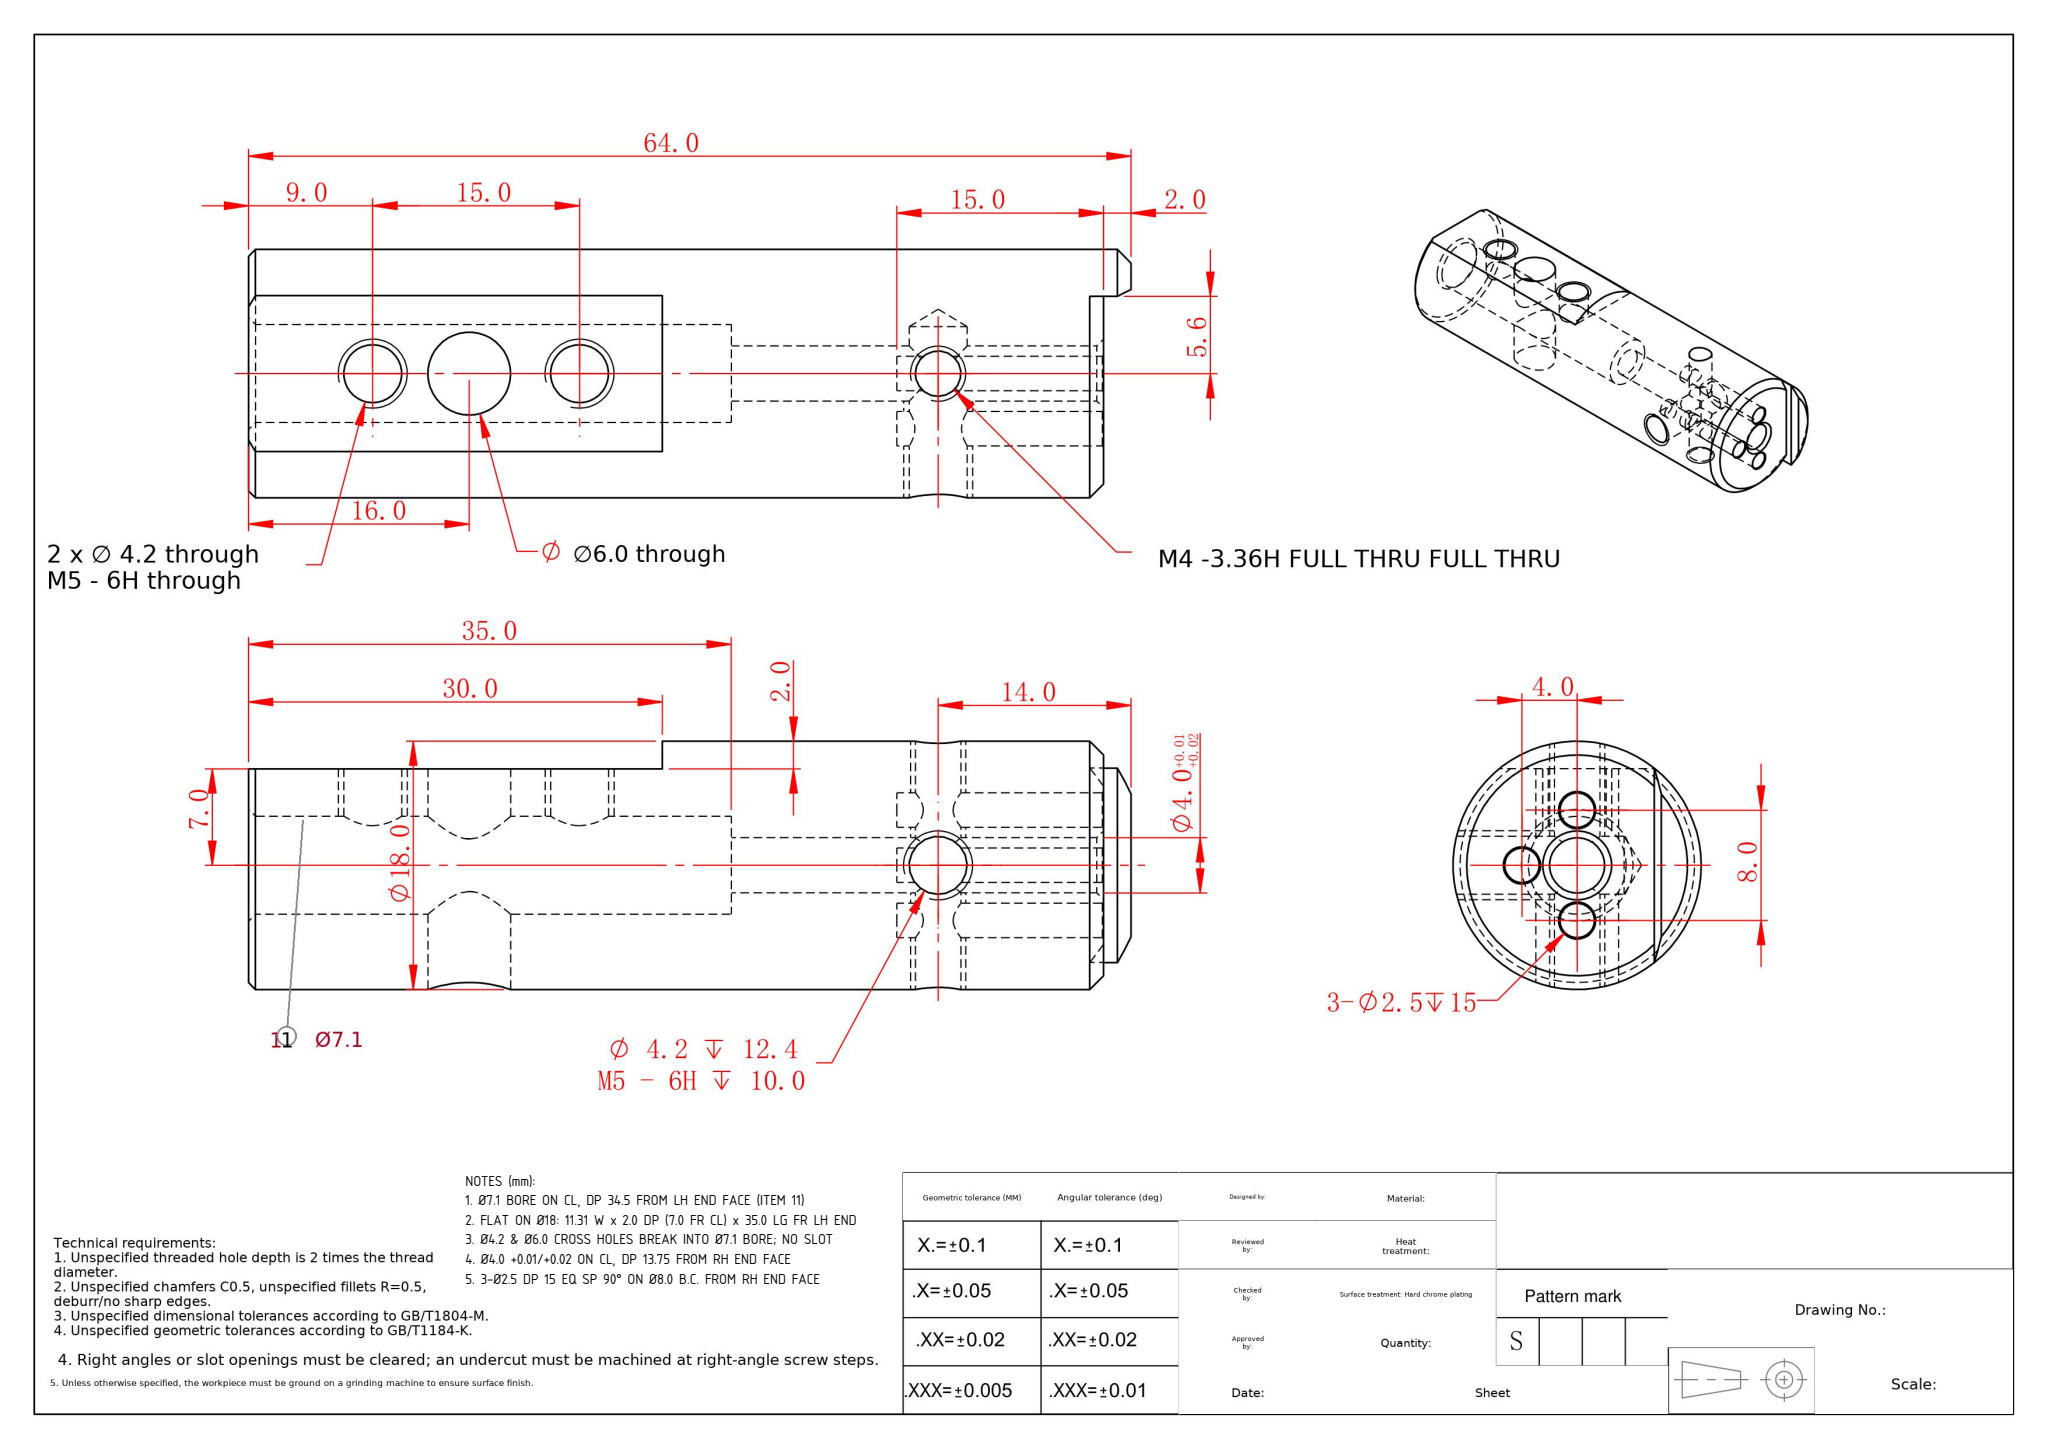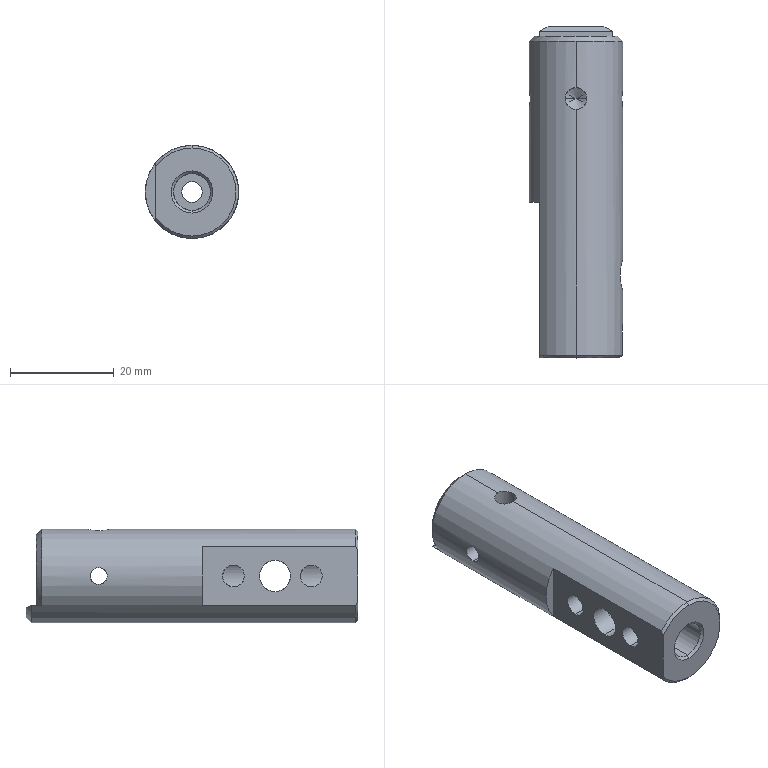Part | SolidWorks | mm | 1 solid | 65 faces | box 18 x 64 x 18 mm | volume 12825 mm3 | cylinder 36 | cone 18 | plane 11 | commonest cylinder face diameters 2.5 x12 4.2 x8 6 x4 3.3 x4 4 x4 7.1 x2 18 x2
Drawing notes:
Ø7.1 BORE ON CL, DP 34.5 FROM LH END FACE (ITEM 11) | from the solid: cylinder dia 7.1 axis y at (x9,z9), length 34.5; bbox y 0-64, LH end = y0 plane
FLAT ON Ø18: 11.31 W x 2.0 DP (7.0 FR CL) x 35.0 LG FR LH END | from the solid: plane normal x at x=2.0 (axis x9 -> 7.0 offset); chord 2*sqrt(9^2-7^2)=11.31; y planes 0 and 35.0
Ø4.2 & Ø6.0 CROSS HOLES BREAK INTO Ø7.1 BORE; NO SLOT | from the solid: x-axis holes Ø4.2 at y9 & y24, Ø6.0 at y16, all z9; no slot faces, fillet_radii empty
Ø4.0 +0.01/+0.02 ON CL, DP 13.75 FROM RH END FACE | from the solid: Ø4.0 y-axis cylinder at (9,9), max face length 13.75, runs y64 to y50.25 at cross holes y=50
3-Ø2.5 DP 15 EQ SP 90° ON Ø8.0 B.C. FROM RH END FACE | from the solid: Ø2.5 y-axis holes at (5,9),(9,13),(13,9) = R4.0 from CL (9,9), 90° apart; y64 end face
build123d program:
from build123d import *

# Parameters (mm, degrees)
SKETCH1_R              = 9
BOSS_EXTRUDE1_DEPTH    = 64
SKETCH2_R              = 3.55
CUT_EXTRUDE1_DEPTH     = 35
CUT_EXTRUDE2_REACH     = 67.253
SKETCH3_R              = 2
SKETCH4_W              = 14.6
SKETCH4_H              = 2
CUT_EXTRUDE3_DEPTH     = 10
CHAMFER2_SIZE          = 1
CHAMFER2_SIZE2         = 0.5
CHAMFER5_SIZE          = 1
CHAMFER6_SIZE          = 0.5
SKETCH5_W              = 4
SKETCH5_H              = 16
CUT_EXTRUDE4_DEPTH     = 30
M5_TAPPED_HOLE1_REACH  = 68.581
M5_TAPPED_HOLE1_BORE_R = 2.1
SKETCH8_R              = 1.25
CUT_EXTRUDE5_DEPTH     = 15
M4_TAPPED_HOLE1_D      = 3.3
M5_TAPPED_HOLE2_D      = 4.2
M5_TAPPED_HOLE2_DEPTH  = 12.4
M5_TAPPED_HOLE2_TIP    = 1.262
CHAMFER7_SIZE          = 0.1
SKETCH13_R             = 3
CUT_EXTRUDE6_DEPTH     = 67.581


with BuildPart() as part:
    # Sketch1 → Boss-Extrude1 (new body)
    with BuildSketch(Plane(origin=(0, 0, 0), x_dir=(1, 0, 0), z_dir=(0, 1, 0))):
        with Locations(Location((0, 0, 0), (0, 0, 270))):
            Circle(SKETCH1_R)
    extrude(amount=BOSS_EXTRUDE1_DEPTH)

    # Sketch2 → Cut-Extrude1 (cut)
    with BuildSketch(Plane.XZ):
        with Locations(Location((0, 0, 0), (0, 0, 270))):
            Circle(SKETCH2_R)
    extrude(amount=-CUT_EXTRUDE1_DEPTH, mode=Mode.SUBTRACT)

    # Sketch3 → Cut-Extrude2 (cut, up to next)
    with BuildSketch(Plane(origin=(0, 64, 0), x_dir=(1, 0, 0), z_dir=(0, 1, 0)), mode=Mode.PRIVATE) as cut_extrude2_sk1:
        with Locations(Location((0, 0, 0), (0, 0, 270))):
            Circle(SKETCH3_R)
    cut_extrude2_tool1 = extrude(cut_extrude2_sk1.sketch, amount=-CUT_EXTRUDE2_REACH, mode=Mode.PRIVATE) & part.part
    add(cut_extrude2_tool1.solids().sort_by_distance((0, 64, 0))[0], mode=Mode.SUBTRACT)

    # Sketch4 → Cut-Extrude3 (cut, symmetric)
    with BuildSketch(Plane(origin=(0, 0, 0), x_dir=(0, 0, -1), z_dir=(1, 0, 0))):
        with Locations((-1.7, 63)):
            Rectangle(SKETCH4_W, SKETCH4_H)
    extrude(amount=CUT_EXTRUDE3_DEPTH, both=True, mode=Mode.SUBTRACT)

    # Chamfer2
    chamfer2_edges = [part.edges().sort_by_distance(p)[0] for p in [
        (0, 64, -5.6),
    ]]
    chamfer2_side = [part.faces().sort_by_distance(p)[0] for p in [
        (0, 63, -5.6),
    ]]
    chamfer(chamfer2_edges, length=CHAMFER2_SIZE, length2=CHAMFER2_SIZE2, reference=chamfer2_side[0])

    # Chamfer5
    chamfer5_edges = [part.edges().sort_by_distance(p)[0] for p in [
        (0, 64, -9),
        (-8.106, 62, 3.912),
    ]]
    chamfer(chamfer5_edges, length=CHAMFER5_SIZE)

    # Chamfer6
    chamfer6_edges = [part.edges().sort_by_distance(p)[0] for p in [
        (0, 0, -9),
        (0, 62, -2),
        (0, 0, 3.55),
    ]]
    chamfer(chamfer6_edges, length=CHAMFER6_SIZE)

    # Sketch5 → Cut-Extrude4 (cut)
    with BuildSketch(Plane.XZ):
        with Locations((-9, 0)):
            Rectangle(SKETCH5_W, SKETCH5_H)
    extrude(amount=-CUT_EXTRUDE4_DEPTH, mode=Mode.SUBTRACT)

    # M5 Tapped Hole1 bore → M5 Tapped Hole1 (cut, up to next)
    with BuildSketch(Plane.ZY.offset(7), mode=Mode.PRIVATE) as m5_tapped_hole1_sk1:
        with Locations((0, 24)):
            Circle(M5_TAPPED_HOLE1_BORE_R)
    m5_tapped_hole1_tool1 = extrude(m5_tapped_hole1_sk1.sketch, amount=-M5_TAPPED_HOLE1_REACH, mode=Mode.PRIVATE) & part.part
    # M5 Tapped Hole1 bore → M5 Tapped Hole1 (cut, up to next)
    with BuildSketch(Plane.ZY.offset(7), mode=Mode.PRIVATE) as m5_tapped_hole1_sk2:
        with Locations((0, 9)):
            Circle(M5_TAPPED_HOLE1_BORE_R)
    m5_tapped_hole1_tool2 = extrude(m5_tapped_hole1_sk2.sketch, amount=-M5_TAPPED_HOLE1_REACH, mode=Mode.PRIVATE) & part.part
    add(m5_tapped_hole1_tool1.solids().sort_by_distance((-7, 24, 0))[0], mode=Mode.SUBTRACT)
    add(m5_tapped_hole1_tool2.solids().sort_by_distance((-7, 9, 0))[0], mode=Mode.SUBTRACT)

    # Sketch8 → Cut-Extrude5 (cut)
    with BuildSketch(Plane(origin=(0, 62, 0), x_dir=(1, 0, 0), z_dir=(0, 1, 0))):
        with Locations(Location((4, 0, 0), (0, 0, 270))):
            Circle(SKETCH8_R)
        with Locations(Location((0, -4, 0), (0, 0, 270))):
            Circle(SKETCH8_R)
        with Locations(Location((-4, 0, 0), (0, 0, 270))):
            Circle(SKETCH8_R)
    extrude(amount=-CUT_EXTRUDE5_DEPTH, mode=Mode.SUBTRACT)

    # M4 Tapped Hole1 (through all)
    with Locations(Plane(origin=(9, 0, 0), x_dir=(0, 0, -1), z_dir=(1, 0, 0))):
        with Locations((0, 50)):
            Hole(M4_TAPPED_HOLE1_D / 2)

    # M5 Tapped Hole2
    with Locations(Plane.XY.offset(9)):
        with Locations((0, 50)):
            Hole(M5_TAPPED_HOLE2_D / 2, depth=M5_TAPPED_HOLE2_DEPTH)
            with Locations((0, 0, -(M5_TAPPED_HOLE2_DEPTH + M5_TAPPED_HOLE2_TIP / 2))):  # 118° drill point
                Cone(0, M5_TAPPED_HOLE2_D / 2, M5_TAPPED_HOLE2_TIP, mode=Mode.SUBTRACT)

    # Chamfer7
    chamfer7_edges = [part.edges().sort_by_distance(p)[0] for p in [
        (4, 62, -1.25),
        (0, 62, 2.75),
        (-4, 62, -1.25),
    ]]
    chamfer(chamfer7_edges, length=CHAMFER7_SIZE)

    # Sketch13 → Cut-Extrude6 (cut, through all)
    with BuildSketch(Plane.ZY.offset(7)):
        with Locations((0, 16)):
            Circle(SKETCH13_R)
    extrude(amount=-CUT_EXTRUDE6_DEPTH, mode=Mode.SUBTRACT)


solid = part.part